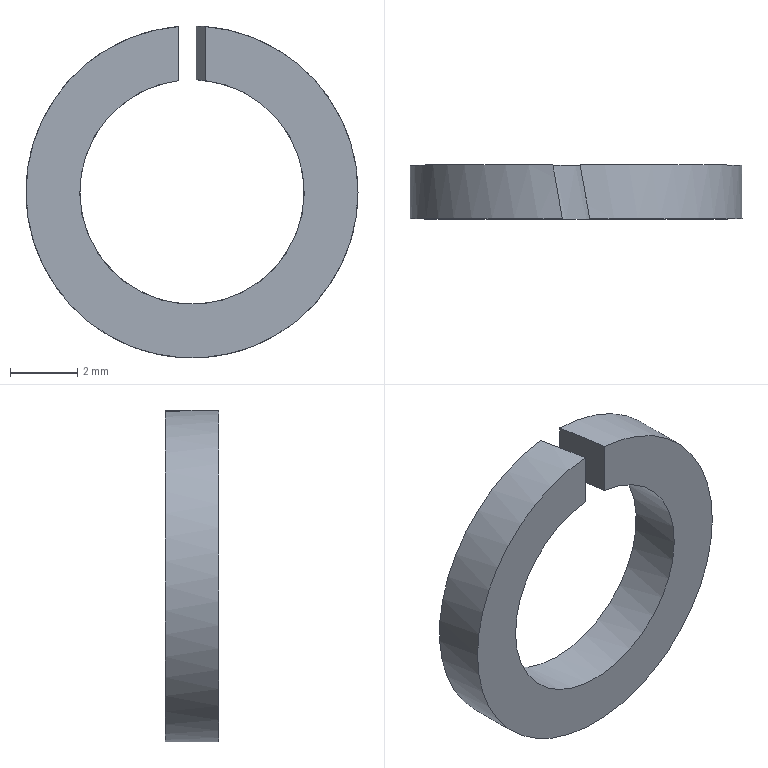Component | NX | SPRING_WASHER_M6_3 | 1 solid | 6 faces | box 9.88 x 1.6 x 9.88 mm | volume 65 mm3 | plane 4 | cylinder 2 | commonest cylinder face diameters 9.88 x1 6.68 x1
STEP:
#1=CARTESIAN_POINT('',(0.,0.,0.));
#2=DIRECTION('',(0.,0.,1.));
#3=DIRECTION('',(1.,0.,0.));
#4=AXIS2_PLACEMENT_3D('',#1,#2,#3);
#5=CARTESIAN_POINT('',(-0.4062,258.,-60.077));
#6=VERTEX_POINT('',#5);
#7=CARTESIAN_POINT('',(0.4062,258.,-60.077));
#8=VERTEX_POINT('',#7);
#9=CARTESIAN_POINT('',(-0.,258.,-65.));
#10=DIRECTION('',(0.,-1.,0.));
#11=DIRECTION('',(0.,0.,-1.));
#12=AXIS2_PLACEMENT_3D('',#9,#10,#11);
#13=CIRCLE('',#12,4.94);
#14=CARTESIAN_POINT('',(-0.,258.,-65.));
#15=DIRECTION('',(0.,-1.,0.));
#16=DIRECTION('',(0.,0.,-1.));
#17=AXIS2_PLACEMENT_3D('',#14,#15,#16);
#18=CYLINDRICAL_SURFACE('',#17,4.94);
#19=CARTESIAN_POINT('',(-6.283,0.));
#20=DIRECTION('',(1.,0.));
#21=VECTOR('',#20,1.);
#22=LINE('',#19,#21);
#23=(GEOMETRIC_REPRESENTATION_CONTEXT(2)PARAMETRIC_REPRESENTATION_CONTEXT()REPRESENTATION_CONTEXT('',''));
#24=DEFINITIONAL_REPRESENTATION('',(#22),#23);
#25=PCURVE('',#18,#24);
#26=CARTESIAN_POINT('',(3.34,258.,-65.));
#27=DIRECTION('',(0.,-1.,0.));
#28=DIRECTION('',(0.,0.,-1.));
#29=AXIS2_PLACEMENT_3D('',#26,#27,#28);
#30=PLANE('',#29);
#31=CARTESIAN_POINT('',(0.,-3.34));
#32=DIRECTION('',(1.,0.));
#33=AXIS2_PLACEMENT_2D('',#31,#32);
#34=CIRCLE('',#33,4.94);
#35=(GEOMETRIC_REPRESENTATION_CONTEXT(2)PARAMETRIC_REPRESENTATION_CONTEXT()REPRESENTATION_CONTEXT('',''));
#36=DEFINITIONAL_REPRESENTATION('',(#34),#35);
#37=PCURVE('',#30,#36);
#38=SURFACE_CURVE('',#13,(#25,#37),.PCURVE_S1.);
#39=EDGE_CURVE('',#6,#8,#38,.T.);
#40=ORIENTED_EDGE('',*,*,#39,.F.);
#41=CARTESIAN_POINT('',(-0.6883,259.6,-60.108));
#42=VERTEX_POINT('',#41);
#43=CARTESIAN_POINT('',(-0.,255.696,-65.));
#44=DIRECTION('',(-0.9848,-0.1736,0.));
#45=DIRECTION('',(0.1736,-0.9848,0.));
#46=AXIS2_PLACEMENT_3D('',#43,#44,#45);
#47=ELLIPSE('',#46,28.448,4.94);
#48=CARTESIAN_POINT('',(-3.059,0.));
#49=CARTESIAN_POINT('',(-3.002,-1.6));
#50=B_SPLINE_CURVE_WITH_KNOTS('',1,(#48,#49),.UNSPECIFIED.,.F.,.F.,(2,2),(1.653,1.711),.PIECEWISE_BEZIER_KNOTS.);
#51=(GEOMETRIC_REPRESENTATION_CONTEXT(2)PARAMETRIC_REPRESENTATION_CONTEXT()REPRESENTATION_CONTEXT('',''));
#52=DEFINITIONAL_REPRESENTATION('',(#50),#51);
#53=PCURVE('',#18,#52);
#54=CARTESIAN_POINT('',(-0.8107,260.294,-57.59));
#55=DIRECTION('',(0.9848,0.1736,0.));
#56=DIRECTION('',(-0.1736,0.9848,0.));
#57=AXIS2_PLACEMENT_3D('',#54,#55,#56);
#58=PLANE('',#57);
#59=CARTESIAN_POINT('',(-33.117,-7.41));
#60=CARTESIAN_POINT('',(-33.117,1.146));
#61=CARTESIAN_POINT('',(9.556,-3.132));
#62=CARTESIAN_POINT('',(52.228,-7.41));
#63=CARTESIAN_POINT('',(9.556,-11.688));
#64=CARTESIAN_POINT('',(-33.117,-15.966));
#65=CARTESIAN_POINT('',(-33.117,-7.41));
#66=(BOUNDED_CURVE()B_SPLINE_CURVE(2,(#59,#60,#61,#62,#63,#64,#65),.UNSPECIFIED.,.T.,.F.)B_SPLINE_CURVE_WITH_KNOTS((1,2,2,2,2,1),(-2.094,0.,2.094,4.189,6.283,8.378),.UNSPECIFIED.)CURVE()GEOMETRIC_REPRESENTATION_ITEM()RATIONAL_B_SPLINE_CURVE((1.,0.5,1.,0.5,1.,0.5,1.))REPRESENTATION_ITEM(''));
#67=(GEOMETRIC_REPRESENTATION_CONTEXT(2)PARAMETRIC_REPRESENTATION_CONTEXT()REPRESENTATION_CONTEXT('',''));
#68=DEFINITIONAL_REPRESENTATION('',(#66),#67);
#69=PCURVE('',#58,#68);
#70=SURFACE_CURVE('',#47,(#53,#69),.PCURVE_S1.);
#71=EDGE_CURVE('',#6,#42,#70,.T.);
#72=ORIENTED_EDGE('',*,*,#71,.T.);
#73=CARTESIAN_POINT('',(0.124,259.6,-60.062));
#74=VERTEX_POINT('',#73);
#75=CARTESIAN_POINT('',(-0.,259.6,-65.));
#76=DIRECTION('',(0.,-1.,0.));
#77=DIRECTION('',(0.,0.,-1.));
#78=AXIS2_PLACEMENT_3D('',#75,#76,#77);
#79=CIRCLE('',#78,4.94);
#80=CARTESIAN_POINT('',(-6.283,-1.6));
#81=DIRECTION('',(1.,0.));
#82=VECTOR('',#81,1.);
#83=LINE('',#80,#82);
#84=(GEOMETRIC_REPRESENTATION_CONTEXT(2)PARAMETRIC_REPRESENTATION_CONTEXT()REPRESENTATION_CONTEXT('',''));
#85=DEFINITIONAL_REPRESENTATION('',(#83),#84);
#86=PCURVE('',#18,#85);
#87=CARTESIAN_POINT('',(4.94,259.6,-65.));
#88=DIRECTION('',(0.,1.,0.));
#89=DIRECTION('',(0.,0.,1.));
#90=AXIS2_PLACEMENT_3D('',#87,#88,#89);
#91=PLANE('',#90);
#92=CARTESIAN_POINT('',(-4.94,-4.94));
#93=CARTESIAN_POINT('',(-4.94,3.616));
#94=CARTESIAN_POINT('',(2.47,-0.6618));
#95=CARTESIAN_POINT('',(9.88,-4.94));
#96=CARTESIAN_POINT('',(2.47,-9.218));
#97=CARTESIAN_POINT('',(-4.94,-13.496));
#98=CARTESIAN_POINT('',(-4.94,-4.94));
#99=(BOUNDED_CURVE()B_SPLINE_CURVE(2,(#92,#93,#94,#95,#96,#97,#98),.UNSPECIFIED.,.T.,.F.)B_SPLINE_CURVE_WITH_KNOTS((1,2,2,2,2,1),(-2.094,0.,2.094,4.189,6.283,8.378),.UNSPECIFIED.)CURVE()GEOMETRIC_REPRESENTATION_ITEM()RATIONAL_B_SPLINE_CURVE((1.,0.5,1.,0.5,1.,0.5,1.))REPRESENTATION_ITEM(''));
#100=(GEOMETRIC_REPRESENTATION_CONTEXT(2)PARAMETRIC_REPRESENTATION_CONTEXT()REPRESENTATION_CONTEXT('',''));
#101=DEFINITIONAL_REPRESENTATION('',(#99),#100);
#102=PCURVE('',#91,#101);
#103=SURFACE_CURVE('',#79,(#86,#102),.PCURVE_S1.);
#104=EDGE_CURVE('',#42,#74,#103,.T.);
#105=ORIENTED_EDGE('',*,*,#104,.T.);
#106=CARTESIAN_POINT('',(-0.,260.304,-65.));
#107=DIRECTION('',(0.9848,0.1736,0.));
#108=DIRECTION('',(0.1736,-0.9848,0.));
#109=AXIS2_PLACEMENT_3D('',#106,#107,#108);
#110=ELLIPSE('',#109,28.448,4.94);
#111=CARTESIAN_POINT('',(3.116,-1.6));
#112=CARTESIAN_POINT('',(3.059,0.));
#113=B_SPLINE_CURVE_WITH_KNOTS('',1,(#111,#112),.UNSPECIFIED.,.F.,.F.,(2,2),(4.738,4.795),.PIECEWISE_BEZIER_KNOTS.);
#114=(GEOMETRIC_REPRESENTATION_CONTEXT(2)PARAMETRIC_REPRESENTATION_CONTEXT()REPRESENTATION_CONTEXT('',''));
#115=DEFINITIONAL_REPRESENTATION('',(#113),#114);
#116=PCURVE('',#18,#115);
#117=CARTESIAN_POINT('',(0.8107,255.706,-57.59));
#118=DIRECTION('',(-0.9848,-0.1736,0.));
#119=DIRECTION('',(0.1736,-0.9848,0.));
#120=AXIS2_PLACEMENT_3D('',#117,#118,#119);
#121=PLANE('',#120);
#122=CARTESIAN_POINT('',(23.78,-7.41));
#123=CARTESIAN_POINT('',(23.78,-15.966));
#124=CARTESIAN_POINT('',(-18.893,-11.688));
#125=CARTESIAN_POINT('',(-61.565,-7.41));
#126=CARTESIAN_POINT('',(-18.893,-3.132));
#127=CARTESIAN_POINT('',(23.78,1.146));
#128=CARTESIAN_POINT('',(23.78,-7.41));
#129=(BOUNDED_CURVE()B_SPLINE_CURVE(2,(#122,#123,#124,#125,#126,#127,#128),.UNSPECIFIED.,.T.,.F.)B_SPLINE_CURVE_WITH_KNOTS((1,2,2,2,2,1),(-2.094,0.,2.094,4.189,6.283,8.378),.UNSPECIFIED.)CURVE()GEOMETRIC_REPRESENTATION_ITEM()RATIONAL_B_SPLINE_CURVE((1.,0.5,1.,0.5,1.,0.5,1.))REPRESENTATION_ITEM(''));
#130=(GEOMETRIC_REPRESENTATION_CONTEXT(2)PARAMETRIC_REPRESENTATION_CONTEXT()REPRESENTATION_CONTEXT('',''));
#131=DEFINITIONAL_REPRESENTATION('',(#129),#130);
#132=PCURVE('',#121,#131);
#133=SURFACE_CURVE('',#110,(#116,#132),.PCURVE_S1.);
#134=EDGE_CURVE('',#74,#8,#133,.T.);
#135=ORIENTED_EDGE('',*,*,#134,.T.);
#136=EDGE_LOOP('',(#40,#72,#105,#135));
#137=FACE_BOUND('',#136,.T.);
#138=ADVANCED_FACE('',(#137),#18,.T.);
#139=ORIENTED_EDGE('',*,*,#104,.F.);
#140=CARTESIAN_POINT('',(-0.6883,259.6,-61.732));
#141=VERTEX_POINT('',#140);
#142=CARTESIAN_POINT('',(-0.6883,259.6,-65.));
#143=DIRECTION('',(0.,0.,-1.));
#144=VECTOR('',#143,1.);
#145=LINE('',#142,#144);
#146=CARTESIAN_POINT('',(0.,-5.628));
#147=DIRECTION('',(-1.,0.));
#148=VECTOR('',#147,1.);
#149=LINE('',#146,#148);
#150=(GEOMETRIC_REPRESENTATION_CONTEXT(2)PARAMETRIC_REPRESENTATION_CONTEXT()REPRESENTATION_CONTEXT('',''));
#151=DEFINITIONAL_REPRESENTATION('',(#149),#150);
#152=PCURVE('',#91,#151);
#153=CARTESIAN_POINT('',(-0.7048,-7.41));
#154=DIRECTION('',(0.,-1.));
#155=VECTOR('',#154,1.);
#156=LINE('',#153,#155);
#157=(GEOMETRIC_REPRESENTATION_CONTEXT(2)PARAMETRIC_REPRESENTATION_CONTEXT()REPRESENTATION_CONTEXT('',''));
#158=DEFINITIONAL_REPRESENTATION('',(#156),#157);
#159=PCURVE('',#58,#158);
#160=SURFACE_CURVE('',#145,(#152,#159),.PCURVE_S1.);
#161=EDGE_CURVE('',#42,#141,#160,.T.);
#162=ORIENTED_EDGE('',*,*,#161,.T.);
#163=CARTESIAN_POINT('',(0.124,259.6,-61.662));
#164=VERTEX_POINT('',#163);
#165=CARTESIAN_POINT('',(-0.,259.6,-65.));
#166=DIRECTION('',(0.,-1.,0.));
#167=DIRECTION('',(0.,0.,-1.));
#168=AXIS2_PLACEMENT_3D('',#165,#166,#167);
#169=CIRCLE('',#168,3.34);
#170=CARTESIAN_POINT('',(-3.34,-4.94));
#171=CARTESIAN_POINT('',(-3.34,0.845));
#172=CARTESIAN_POINT('',(1.67,-2.047));
#173=CARTESIAN_POINT('',(6.68,-4.94));
#174=CARTESIAN_POINT('',(1.67,-7.833));
#175=CARTESIAN_POINT('',(-3.34,-10.725));
#176=CARTESIAN_POINT('',(-3.34,-4.94));
#177=(BOUNDED_CURVE()B_SPLINE_CURVE(2,(#170,#171,#172,#173,#174,#175,#176),.UNSPECIFIED.,.T.,.F.)B_SPLINE_CURVE_WITH_KNOTS((1,2,2,2,2,1),(-2.094,0.,2.094,4.189,6.283,8.378),.UNSPECIFIED.)CURVE()GEOMETRIC_REPRESENTATION_ITEM()RATIONAL_B_SPLINE_CURVE((1.,0.5,1.,0.5,1.,0.5,1.))REPRESENTATION_ITEM(''));
#178=(GEOMETRIC_REPRESENTATION_CONTEXT(2)PARAMETRIC_REPRESENTATION_CONTEXT()REPRESENTATION_CONTEXT('',''));
#179=DEFINITIONAL_REPRESENTATION('',(#177),#178);
#180=PCURVE('',#91,#179);
#181=CARTESIAN_POINT('',(-0.,258.,-65.));
#182=DIRECTION('',(0.,-1.,0.));
#183=DIRECTION('',(0.,0.,-1.));
#184=AXIS2_PLACEMENT_3D('',#181,#182,#183);
#185=CYLINDRICAL_SURFACE('',#184,3.34);
#186=CARTESIAN_POINT('',(-6.283,-1.6));
#187=DIRECTION('',(1.,0.));
#188=VECTOR('',#187,1.);
#189=LINE('',#186,#188);
#190=(GEOMETRIC_REPRESENTATION_CONTEXT(2)PARAMETRIC_REPRESENTATION_CONTEXT()REPRESENTATION_CONTEXT('',''));
#191=DEFINITIONAL_REPRESENTATION('',(#189),#190);
#192=PCURVE('',#185,#191);
#193=SURFACE_CURVE('',#169,(#180,#192),.PCURVE_S1.);
#194=EDGE_CURVE('',#141,#164,#193,.T.);
#195=ORIENTED_EDGE('',*,*,#194,.T.);
#196=CARTESIAN_POINT('',(0.124,259.6,-65.));
#197=DIRECTION('',(0.,0.,1.));
#198=VECTOR('',#197,1.);
#199=LINE('',#196,#198);
#200=CARTESIAN_POINT('',(0.,-4.816));
#201=DIRECTION('',(1.,0.));
#202=VECTOR('',#201,1.);
#203=LINE('',#200,#202);
#204=(GEOMETRIC_REPRESENTATION_CONTEXT(2)PARAMETRIC_REPRESENTATION_CONTEXT()REPRESENTATION_CONTEXT('',''));
#205=DEFINITIONAL_REPRESENTATION('',(#203),#204);
#206=PCURVE('',#91,#205);
#207=CARTESIAN_POINT('',(-3.954,-7.41));
#208=DIRECTION('',(0.,1.));
#209=VECTOR('',#208,1.);
#210=LINE('',#207,#209);
#211=(GEOMETRIC_REPRESENTATION_CONTEXT(2)PARAMETRIC_REPRESENTATION_CONTEXT()REPRESENTATION_CONTEXT('',''));
#212=DEFINITIONAL_REPRESENTATION('',(#210),#211);
#213=PCURVE('',#121,#212);
#214=SURFACE_CURVE('',#199,(#206,#213),.PCURVE_S1.);
#215=EDGE_CURVE('',#164,#74,#214,.T.);
#216=ORIENTED_EDGE('',*,*,#215,.T.);
#217=EDGE_LOOP('',(#139,#162,#195,#216));
#218=FACE_BOUND('',#217,.T.);
#219=ADVANCED_FACE('',(#218),#91,.T.);
#220=CARTESIAN_POINT('',(0.4062,258.,-61.685));
#221=VERTEX_POINT('',#220);
#222=CARTESIAN_POINT('',(-0.,260.304,-65.));
#223=DIRECTION('',(-0.9848,-0.1736,0.));
#224=DIRECTION('',(0.1736,-0.9848,0.));
#225=AXIS2_PLACEMENT_3D('',#222,#223,#224);
#226=ELLIPSE('',#225,19.234,3.34);
#227=CARTESIAN_POINT('',(3.02,0.));
#228=CARTESIAN_POINT('',(3.104,-1.6));
#229=B_SPLINE_CURVE_WITH_KNOTS('',1,(#227,#228),.UNSPECIFIED.,.F.,.F.,(2,2),(1.449,1.534),.PIECEWISE_BEZIER_KNOTS.);
#230=(GEOMETRIC_REPRESENTATION_CONTEXT(2)PARAMETRIC_REPRESENTATION_CONTEXT()REPRESENTATION_CONTEXT('',''));
#231=DEFINITIONAL_REPRESENTATION('',(#229),#230);
#232=PCURVE('',#185,#231);
#233=CARTESIAN_POINT('',(-4.669,-7.41));
#234=DIRECTION('',(1.,0.));
#235=AXIS2_PLACEMENT_2D('',#233,#234);
#236=ELLIPSE('',#235,19.234,3.34);
#237=(GEOMETRIC_REPRESENTATION_CONTEXT(2)PARAMETRIC_REPRESENTATION_CONTEXT()REPRESENTATION_CONTEXT('',''));
#238=DEFINITIONAL_REPRESENTATION('',(#236),#237);
#239=PCURVE('',#121,#238);
#240=SURFACE_CURVE('',#226,(#232,#239),.PCURVE_S1.);
#241=EDGE_CURVE('',#221,#164,#240,.T.);
#242=ORIENTED_EDGE('',*,*,#241,.F.);
#243=CARTESIAN_POINT('',(-0.4062,258.,-61.685));
#244=VERTEX_POINT('',#243);
#245=CARTESIAN_POINT('',(-0.,258.,-65.));
#246=DIRECTION('',(0.,-1.,0.));
#247=DIRECTION('',(0.,0.,-1.));
#248=AXIS2_PLACEMENT_3D('',#245,#246,#247);
#249=CIRCLE('',#248,3.34);
#250=CARTESIAN_POINT('',(-6.283,0.));
#251=DIRECTION('',(1.,0.));
#252=VECTOR('',#251,1.);
#253=LINE('',#250,#252);
#254=(GEOMETRIC_REPRESENTATION_CONTEXT(2)PARAMETRIC_REPRESENTATION_CONTEXT()REPRESENTATION_CONTEXT('',''));
#255=DEFINITIONAL_REPRESENTATION('',(#253),#254);
#256=PCURVE('',#185,#255);
#257=CARTESIAN_POINT('',(0.,-3.34));
#258=DIRECTION('',(1.,0.));
#259=AXIS2_PLACEMENT_2D('',#257,#258);
#260=CIRCLE('',#259,3.34);
#261=(GEOMETRIC_REPRESENTATION_CONTEXT(2)PARAMETRIC_REPRESENTATION_CONTEXT()REPRESENTATION_CONTEXT('',''));
#262=DEFINITIONAL_REPRESENTATION('',(#260),#261);
#263=PCURVE('',#30,#262);
#264=SURFACE_CURVE('',#249,(#256,#263),.PCURVE_S1.);
#265=EDGE_CURVE('',#244,#221,#264,.T.);
#266=ORIENTED_EDGE('',*,*,#265,.F.);
#267=CARTESIAN_POINT('',(-0.,255.696,-65.));
#268=DIRECTION('',(0.9848,0.1736,0.));
#269=DIRECTION('',(0.1736,-0.9848,0.));
#270=AXIS2_PLACEMENT_3D('',#267,#268,#269);
#271=ELLIPSE('',#270,19.234,3.34);
#272=CARTESIAN_POINT('',(-2.934,-1.6));
#273=CARTESIAN_POINT('',(-3.02,0.));
#274=B_SPLINE_CURVE_WITH_KNOTS('',1,(#272,#273),.UNSPECIFIED.,.F.,.F.,(2,2),(4.505,4.59),.PIECEWISE_BEZIER_KNOTS.);
#275=(GEOMETRIC_REPRESENTATION_CONTEXT(2)PARAMETRIC_REPRESENTATION_CONTEXT()REPRESENTATION_CONTEXT('',''));
#276=DEFINITIONAL_REPRESENTATION('',(#274),#275);
#277=PCURVE('',#185,#276);
#278=CARTESIAN_POINT('',(-4.669,-7.41));
#279=DIRECTION('',(-1.,0.));
#280=AXIS2_PLACEMENT_2D('',#278,#279);
#281=ELLIPSE('',#280,19.234,3.34);
#282=(GEOMETRIC_REPRESENTATION_CONTEXT(2)PARAMETRIC_REPRESENTATION_CONTEXT()REPRESENTATION_CONTEXT('',''));
#283=DEFINITIONAL_REPRESENTATION('',(#281),#282);
#284=PCURVE('',#58,#283);
#285=SURFACE_CURVE('',#271,(#277,#284),.PCURVE_S1.);
#286=EDGE_CURVE('',#141,#244,#285,.T.);
#287=ORIENTED_EDGE('',*,*,#286,.F.);
#288=ORIENTED_EDGE('',*,*,#194,.T.);
#289=EDGE_LOOP('',(#242,#266,#287,#288));
#290=FACE_BOUND('',#289,.F.);
#291=ADVANCED_FACE('',(#290),#185,.F.);
#292=ORIENTED_EDGE('',*,*,#265,.F.);
#293=CARTESIAN_POINT('',(-0.4062,258.,-65.));
#294=DIRECTION('',(0.,0.,1.));
#295=VECTOR('',#294,1.);
#296=LINE('',#293,#295);
#297=CARTESIAN_POINT('',(0.,-3.746));
#298=DIRECTION('',(-1.,0.));
#299=VECTOR('',#298,1.);
#300=LINE('',#297,#299);
#301=(GEOMETRIC_REPRESENTATION_CONTEXT(2)PARAMETRIC_REPRESENTATION_CONTEXT()REPRESENTATION_CONTEXT('',''));
#302=DEFINITIONAL_REPRESENTATION('',(#300),#301);
#303=PCURVE('',#30,#302);
#304=CARTESIAN_POINT('',(-2.329,-7.41));
#305=DIRECTION('',(0.,1.));
#306=VECTOR('',#305,1.);
#307=LINE('',#304,#306);
#308=(GEOMETRIC_REPRESENTATION_CONTEXT(2)PARAMETRIC_REPRESENTATION_CONTEXT()REPRESENTATION_CONTEXT('',''));
#309=DEFINITIONAL_REPRESENTATION('',(#307),#308);
#310=PCURVE('',#58,#309);
#311=SURFACE_CURVE('',#296,(#303,#310),.PCURVE_S1.);
#312=EDGE_CURVE('',#244,#6,#311,.T.);
#313=ORIENTED_EDGE('',*,*,#312,.T.);
#314=ORIENTED_EDGE('',*,*,#39,.T.);
#315=CARTESIAN_POINT('',(0.4062,258.,-65.));
#316=DIRECTION('',(0.,0.,-1.));
#317=VECTOR('',#316,1.);
#318=LINE('',#315,#317);
#319=CARTESIAN_POINT('',(0.,-2.934));
#320=DIRECTION('',(1.,0.));
#321=VECTOR('',#320,1.);
#322=LINE('',#319,#321);
#323=(GEOMETRIC_REPRESENTATION_CONTEXT(2)PARAMETRIC_REPRESENTATION_CONTEXT()REPRESENTATION_CONTEXT('',''));
#324=DEFINITIONAL_REPRESENTATION('',(#322),#323);
#325=PCURVE('',#30,#324);
#326=CARTESIAN_POINT('',(-2.329,-7.41));
#327=DIRECTION('',(0.,-1.));
#328=VECTOR('',#327,1.);
#329=LINE('',#326,#328);
#330=(GEOMETRIC_REPRESENTATION_CONTEXT(2)PARAMETRIC_REPRESENTATION_CONTEXT()REPRESENTATION_CONTEXT('',''));
#331=DEFINITIONAL_REPRESENTATION('',(#329),#330);
#332=PCURVE('',#121,#331);
#333=SURFACE_CURVE('',#318,(#325,#332),.PCURVE_S1.);
#334=EDGE_CURVE('',#8,#221,#333,.T.);
#335=ORIENTED_EDGE('',*,*,#334,.T.);
#336=EDGE_LOOP('',(#292,#313,#314,#335));
#337=FACE_BOUND('',#336,.T.);
#338=ADVANCED_FACE('',(#337),#30,.T.);
#339=ORIENTED_EDGE('',*,*,#215,.F.);
#340=ORIENTED_EDGE('',*,*,#241,.F.);
#341=ORIENTED_EDGE('',*,*,#334,.F.);
#342=ORIENTED_EDGE('',*,*,#134,.F.);
#343=EDGE_LOOP('',(#339,#340,#341,#342));
#344=FACE_BOUND('',#343,.T.);
#345=ADVANCED_FACE('',(#344),#121,.T.);
#346=ORIENTED_EDGE('',*,*,#312,.F.);
#347=ORIENTED_EDGE('',*,*,#286,.F.);
#348=ORIENTED_EDGE('',*,*,#161,.F.);
#349=ORIENTED_EDGE('',*,*,#71,.F.);
#350=EDGE_LOOP('',(#346,#347,#348,#349));
#351=FACE_BOUND('',#350,.T.);
#352=ADVANCED_FACE('',(#351),#58,.T.);
#353=CLOSED_SHELL('',(#138,#219,#291,#338,#345,#352));
#354=MANIFOLD_SOLID_BREP('',#353);
#355=(LENGTH_UNIT()NAMED_UNIT(*)SI_UNIT(.MILLI.,.METRE.));
#356=UNCERTAINTY_MEASURE_WITH_UNIT(LENGTH_MEASURE(0.001),#355,'','');
#357=(NAMED_UNIT(*)PLANE_ANGLE_UNIT()SI_UNIT($,.RADIAN.));
#358=(NAMED_UNIT(*)SI_UNIT($,.STERADIAN.)SOLID_ANGLE_UNIT());
#359=(GEOMETRIC_REPRESENTATION_CONTEXT(3)GLOBAL_UNCERTAINTY_ASSIGNED_CONTEXT((#356))GLOBAL_UNIT_ASSIGNED_CONTEXT((#355,#357,#358))REPRESENTATION_CONTEXT('',''));
#360=ADVANCED_BREP_SHAPE_REPRESENTATION('',(#4,#354),#359);